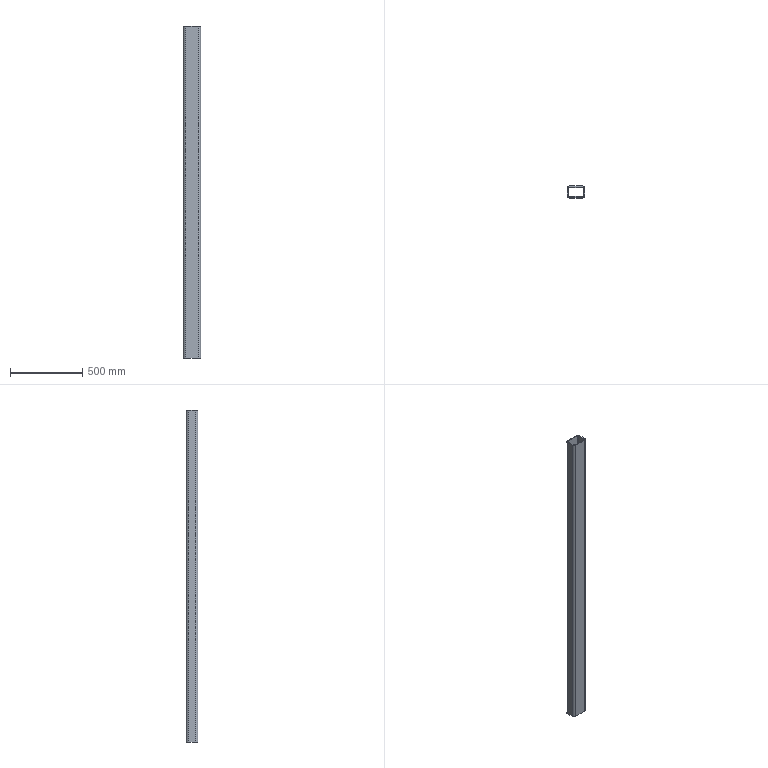Component | SolidWorks | ST60-04-1 | 1 solid | 18 faces | box 120 x 80 x 2300 mm | volume 6392127 mm3 | plane 10 | cylinder 8 | commonest cylinder face diameters 32 x4 16 x4
build123d program:
from build123d import *

# Parameters (mm, degrees)
RECTANGULAR_TUBE_120_X_80_X_8_1_DEPTH = 2300


with BuildPart() as part:
    # Sketch1 → Rectangular Tube 120 X 80 X 8_1 (new body)
    with BuildSketch(Plane.YZ):
        with BuildLine():
            Line((-24, -60), (24, -60))
            ThreePointArc((24, -60), (35.314, -55.314), (40, -44))
            Line((40, -44), (40, 44))
            ThreePointArc((40, 44), (35.314, 55.314), (24, 60))
            Line((24, 60), (-24, 60))
            ThreePointArc((-24, 60), (-35.314, 55.314), (-40, 44))
            Line((-40, 44), (-40, -44))
            ThreePointArc((-40, -44), (-35.314, -55.314), (-24, -60))
        make_face()
        with BuildLine():
            Line((-24, -52), (24, -52))
            ThreePointArc((24, -52), (29.657, -49.657), (32, -44))
            Line((32, -44), (32, 44))
            ThreePointArc((32, 44), (29.657, 49.657), (24, 52))
            Line((24, 52), (-24, 52))
            ThreePointArc((-24, 52), (-29.657, 49.657), (-32, 44))
            Line((-32, 44), (-32, -44))
            ThreePointArc((-32, -44), (-29.657, -49.657), (-24, -52))
        make_face(mode=Mode.SUBTRACT)
    extrude(amount=RECTANGULAR_TUBE_120_X_80_X_8_1_DEPTH)


solid = part.part

# Placed as in the assembly
solid = solid.moved(Location((592.993, -4.546, -60), (0, 90, 0)))
STEP:
#1=COLOUR_RGB('',0.7922,0.8196,0.9333);
#2=FILL_AREA_STYLE_COLOUR('',#1);
#3=FILL_AREA_STYLE('',(#2));
#4=SURFACE_STYLE_FILL_AREA(#3);
#5=SURFACE_SIDE_STYLE('',(#4));
#6=SURFACE_STYLE_USAGE(.BOTH.,#5);
#7=PRESENTATION_STYLE_ASSIGNMENT((#6));
#8=CARTESIAN_POINT('',(21.614,1.396,-92.913));
#9=VERTEX_POINT('',#8);
#10=CARTESIAN_POINT('',(20.984,0.7659,-92.913));
#11=VERTEX_POINT('',#10);
#12=CARTESIAN_POINT('',(21.614,0.7659,-92.913));
#13=DIRECTION('',(0.,0.,1.));
#14=DIRECTION('',(1.,0.,0.));
#15=AXIS2_PLACEMENT_3D('',#12,#13,#14);
#16=CIRCLE('',#15,0.6299);
#17=EDGE_CURVE('',#9,#11,#16,.T.);
#18=ORIENTED_EDGE('',*,*,#17,.T.);
#19=CARTESIAN_POINT('',(20.984,0.7659,-2.362));
#20=VERTEX_POINT('',#19);
#21=CARTESIAN_POINT('',(20.984,0.7659,-2.362));
#22=DIRECTION('',(0.,0.,-1.));
#23=VECTOR('',#22,39.37);
#24=LINE('',#21,#23);
#25=EDGE_CURVE('',#20,#11,#24,.T.);
#26=ORIENTED_EDGE('',*,*,#25,.F.);
#27=CARTESIAN_POINT('',(21.614,1.396,-2.362));
#28=VERTEX_POINT('',#27);
#29=CARTESIAN_POINT('',(21.614,0.7659,-2.362));
#30=DIRECTION('',(0.,0.,1.));
#31=DIRECTION('',(1.,0.,0.));
#32=AXIS2_PLACEMENT_3D('',#29,#30,#31);
#33=CIRCLE('',#32,0.6299);
#34=EDGE_CURVE('',#28,#20,#33,.T.);
#35=ORIENTED_EDGE('',*,*,#34,.F.);
#36=CARTESIAN_POINT('',(21.614,1.396,-2.362));
#37=DIRECTION('',(0.,0.,-1.));
#38=VECTOR('',#37,39.37);
#39=LINE('',#36,#38);
#40=EDGE_CURVE('',#28,#9,#39,.T.);
#41=ORIENTED_EDGE('',*,*,#40,.T.);
#42=EDGE_LOOP('',(#18,#26,#35,#41));
#43=FACE_OUTER_BOUND('',#42,.T.);
#44=CARTESIAN_POINT('',(21.614,0.7659,-2.362));
#45=DIRECTION('',(0.,0.,-1.));
#46=DIRECTION('',(-1.,0.,0.));
#47=AXIS2_PLACEMENT_3D('',#44,#45,#46);
#48=CYLINDRICAL_SURFACE('',#47,0.6299);
#49=ADVANCED_FACE('',(#43),#48,.T.);
#50=CARTESIAN_POINT('',(20.984,-1.124,-92.913));
#51=VERTEX_POINT('',#50);
#52=CARTESIAN_POINT('',(20.984,0.7659,-92.913));
#53=DIRECTION('',(0.,-1.,0.));
#54=VECTOR('',#53,39.37);
#55=LINE('',#52,#54);
#56=EDGE_CURVE('',#11,#51,#55,.T.);
#57=ORIENTED_EDGE('',*,*,#56,.T.);
#58=CARTESIAN_POINT('',(20.984,-1.124,-2.362));
#59=VERTEX_POINT('',#58);
#60=CARTESIAN_POINT('',(20.984,-1.124,-2.362));
#61=DIRECTION('',(0.,0.,-1.));
#62=VECTOR('',#61,39.37);
#63=LINE('',#60,#62);
#64=EDGE_CURVE('',#59,#51,#63,.T.);
#65=ORIENTED_EDGE('',*,*,#64,.F.);
#66=CARTESIAN_POINT('',(20.984,0.7659,-2.362));
#67=DIRECTION('',(0.,-1.,0.));
#68=VECTOR('',#67,39.37);
#69=LINE('',#66,#68);
#70=EDGE_CURVE('',#20,#59,#69,.T.);
#71=ORIENTED_EDGE('',*,*,#70,.F.);
#72=ORIENTED_EDGE('',*,*,#25,.T.);
#73=EDGE_LOOP('',(#57,#65,#71,#72));
#74=FACE_OUTER_BOUND('',#73,.T.);
#75=CARTESIAN_POINT('',(20.984,0.7659,-2.362));
#76=DIRECTION('',(1.,0.,0.));
#77=DIRECTION('',(0.,0.,-1.));
#78=AXIS2_PLACEMENT_3D('',#75,#76,#77);
#79=PLANE('',#78);
#80=ADVANCED_FACE('',(#74),#79,.F.);
#81=CARTESIAN_POINT('',(21.614,-1.754,-92.913));
#82=VERTEX_POINT('',#81);
#83=CARTESIAN_POINT('',(21.614,-1.124,-92.913));
#84=DIRECTION('',(0.,0.,1.));
#85=DIRECTION('',(1.,0.,0.));
#86=AXIS2_PLACEMENT_3D('',#83,#84,#85);
#87=CIRCLE('',#86,0.6299);
#88=EDGE_CURVE('',#51,#82,#87,.T.);
#89=ORIENTED_EDGE('',*,*,#88,.T.);
#90=CARTESIAN_POINT('',(21.614,-1.754,-2.362));
#91=VERTEX_POINT('',#90);
#92=CARTESIAN_POINT('',(21.614,-1.754,-2.362));
#93=DIRECTION('',(0.,0.,-1.));
#94=VECTOR('',#93,39.37);
#95=LINE('',#92,#94);
#96=EDGE_CURVE('',#91,#82,#95,.T.);
#97=ORIENTED_EDGE('',*,*,#96,.F.);
#98=CARTESIAN_POINT('',(21.614,-1.124,-2.362));
#99=DIRECTION('',(0.,0.,1.));
#100=DIRECTION('',(1.,0.,0.));
#101=AXIS2_PLACEMENT_3D('',#98,#99,#100);
#102=CIRCLE('',#101,0.6299);
#103=EDGE_CURVE('',#59,#91,#102,.T.);
#104=ORIENTED_EDGE('',*,*,#103,.F.);
#105=ORIENTED_EDGE('',*,*,#64,.T.);
#106=EDGE_LOOP('',(#89,#97,#104,#105));
#107=FACE_OUTER_BOUND('',#106,.T.);
#108=CARTESIAN_POINT('',(21.614,-1.124,-2.362));
#109=DIRECTION('',(0.,0.,-1.));
#110=DIRECTION('',(-1.,0.,0.));
#111=AXIS2_PLACEMENT_3D('',#108,#109,#110);
#112=CYLINDRICAL_SURFACE('',#111,0.6299);
#113=ADVANCED_FACE('',(#107),#112,.T.);
#114=CARTESIAN_POINT('',(25.078,-1.754,-92.913));
#115=VERTEX_POINT('',#114);
#116=CARTESIAN_POINT('',(25.078,-1.754,-92.913));
#117=DIRECTION('',(1.,0.,0.));
#118=VECTOR('',#117,39.37);
#119=LINE('',#116,#118);
#120=EDGE_CURVE('',#82,#115,#119,.T.);
#121=ORIENTED_EDGE('',*,*,#120,.T.);
#122=CARTESIAN_POINT('',(25.078,-1.754,-2.362));
#123=VERTEX_POINT('',#122);
#124=CARTESIAN_POINT('',(25.078,-1.754,-2.362));
#125=DIRECTION('',(0.,0.,-1.));
#126=VECTOR('',#125,39.37);
#127=LINE('',#124,#126);
#128=EDGE_CURVE('',#123,#115,#127,.T.);
#129=ORIENTED_EDGE('',*,*,#128,.F.);
#130=CARTESIAN_POINT('',(25.078,-1.754,-2.362));
#131=DIRECTION('',(1.,0.,0.));
#132=VECTOR('',#131,39.37);
#133=LINE('',#130,#132);
#134=EDGE_CURVE('',#91,#123,#133,.T.);
#135=ORIENTED_EDGE('',*,*,#134,.F.);
#136=ORIENTED_EDGE('',*,*,#96,.T.);
#137=EDGE_LOOP('',(#121,#129,#135,#136));
#138=FACE_OUTER_BOUND('',#137,.T.);
#139=CARTESIAN_POINT('',(25.078,-1.754,-2.362));
#140=DIRECTION('',(0.,1.,0.));
#141=DIRECTION('',(-1.,0.,0.));
#142=AXIS2_PLACEMENT_3D('',#139,#140,#141);
#143=PLANE('',#142);
#144=ADVANCED_FACE('',(#138),#143,.F.);
#145=CARTESIAN_POINT('',(25.708,-1.124,-92.913));
#146=VERTEX_POINT('',#145);
#147=CARTESIAN_POINT('',(25.078,-1.124,-92.913));
#148=DIRECTION('',(0.,0.,1.));
#149=DIRECTION('',(1.,0.,0.));
#150=AXIS2_PLACEMENT_3D('',#147,#148,#149);
#151=CIRCLE('',#150,0.6299);
#152=EDGE_CURVE('',#115,#146,#151,.T.);
#153=ORIENTED_EDGE('',*,*,#152,.T.);
#154=CARTESIAN_POINT('',(25.708,-1.124,-2.362));
#155=VERTEX_POINT('',#154);
#156=CARTESIAN_POINT('',(25.708,-1.124,-2.362));
#157=DIRECTION('',(0.,0.,-1.));
#158=VECTOR('',#157,39.37);
#159=LINE('',#156,#158);
#160=EDGE_CURVE('',#155,#146,#159,.T.);
#161=ORIENTED_EDGE('',*,*,#160,.F.);
#162=CARTESIAN_POINT('',(25.078,-1.124,-2.362));
#163=DIRECTION('',(0.,0.,1.));
#164=DIRECTION('',(1.,0.,0.));
#165=AXIS2_PLACEMENT_3D('',#162,#163,#164);
#166=CIRCLE('',#165,0.6299);
#167=EDGE_CURVE('',#123,#155,#166,.T.);
#168=ORIENTED_EDGE('',*,*,#167,.F.);
#169=ORIENTED_EDGE('',*,*,#128,.T.);
#170=EDGE_LOOP('',(#153,#161,#168,#169));
#171=FACE_OUTER_BOUND('',#170,.T.);
#172=CARTESIAN_POINT('',(25.078,-1.124,-2.362));
#173=DIRECTION('',(0.,0.,-1.));
#174=DIRECTION('',(-1.,0.,0.));
#175=AXIS2_PLACEMENT_3D('',#172,#173,#174);
#176=CYLINDRICAL_SURFACE('',#175,0.6299);
#177=ADVANCED_FACE('',(#171),#176,.T.);
#178=CARTESIAN_POINT('',(25.708,0.7659,-92.913));
#179=VERTEX_POINT('',#178);
#180=CARTESIAN_POINT('',(25.708,-1.124,-92.913));
#181=DIRECTION('',(0.,1.,0.));
#182=VECTOR('',#181,39.37);
#183=LINE('',#180,#182);
#184=EDGE_CURVE('',#146,#179,#183,.T.);
#185=ORIENTED_EDGE('',*,*,#184,.T.);
#186=CARTESIAN_POINT('',(25.708,0.7659,-2.362));
#187=VERTEX_POINT('',#186);
#188=CARTESIAN_POINT('',(25.708,0.7659,-2.362));
#189=DIRECTION('',(0.,0.,-1.));
#190=VECTOR('',#189,39.37);
#191=LINE('',#188,#190);
#192=EDGE_CURVE('',#187,#179,#191,.T.);
#193=ORIENTED_EDGE('',*,*,#192,.F.);
#194=CARTESIAN_POINT('',(25.708,-1.124,-2.362));
#195=DIRECTION('',(0.,1.,0.));
#196=VECTOR('',#195,39.37);
#197=LINE('',#194,#196);
#198=EDGE_CURVE('',#155,#187,#197,.T.);
#199=ORIENTED_EDGE('',*,*,#198,.F.);
#200=ORIENTED_EDGE('',*,*,#160,.T.);
#201=EDGE_LOOP('',(#185,#193,#199,#200));
#202=FACE_OUTER_BOUND('',#201,.T.);
#203=CARTESIAN_POINT('',(25.708,-1.124,-2.362));
#204=DIRECTION('',(-1.,0.,0.));
#205=DIRECTION('',(0.,0.,1.));
#206=AXIS2_PLACEMENT_3D('',#203,#204,#205);
#207=PLANE('',#206);
#208=ADVANCED_FACE('',(#202),#207,.F.);
#209=CARTESIAN_POINT('',(25.078,1.396,-92.913));
#210=VERTEX_POINT('',#209);
#211=CARTESIAN_POINT('',(25.078,0.7659,-92.913));
#212=DIRECTION('',(0.,0.,1.));
#213=DIRECTION('',(1.,0.,0.));
#214=AXIS2_PLACEMENT_3D('',#211,#212,#213);
#215=CIRCLE('',#214,0.6299);
#216=EDGE_CURVE('',#179,#210,#215,.T.);
#217=ORIENTED_EDGE('',*,*,#216,.T.);
#218=CARTESIAN_POINT('',(25.078,1.396,-2.362));
#219=VERTEX_POINT('',#218);
#220=CARTESIAN_POINT('',(25.078,1.396,-2.362));
#221=DIRECTION('',(0.,0.,-1.));
#222=VECTOR('',#221,39.37);
#223=LINE('',#220,#222);
#224=EDGE_CURVE('',#219,#210,#223,.T.);
#225=ORIENTED_EDGE('',*,*,#224,.F.);
#226=CARTESIAN_POINT('',(25.078,0.7659,-2.362));
#227=DIRECTION('',(0.,0.,1.));
#228=DIRECTION('',(1.,0.,0.));
#229=AXIS2_PLACEMENT_3D('',#226,#227,#228);
#230=CIRCLE('',#229,0.6299);
#231=EDGE_CURVE('',#187,#219,#230,.T.);
#232=ORIENTED_EDGE('',*,*,#231,.F.);
#233=ORIENTED_EDGE('',*,*,#192,.T.);
#234=EDGE_LOOP('',(#217,#225,#232,#233));
#235=FACE_OUTER_BOUND('',#234,.T.);
#236=CARTESIAN_POINT('',(25.078,0.7659,-2.362));
#237=DIRECTION('',(0.,0.,-1.));
#238=DIRECTION('',(-1.,0.,0.));
#239=AXIS2_PLACEMENT_3D('',#236,#237,#238);
#240=CYLINDRICAL_SURFACE('',#239,0.6299);
#241=ADVANCED_FACE('',(#235),#240,.T.);
#242=CARTESIAN_POINT('',(21.299,-1.124,-92.913));
#243=VERTEX_POINT('',#242);
#244=CARTESIAN_POINT('',(21.614,-1.439,-92.913));
#245=VERTEX_POINT('',#244);
#246=CARTESIAN_POINT('',(21.614,-1.124,-92.913));
#247=DIRECTION('',(0.,0.,1.));
#248=DIRECTION('',(1.,0.,0.));
#249=AXIS2_PLACEMENT_3D('',#246,#247,#248);
#250=CIRCLE('',#249,0.315);
#251=EDGE_CURVE('',#243,#245,#250,.T.);
#252=ORIENTED_EDGE('',*,*,#251,.F.);
#253=CARTESIAN_POINT('',(21.299,-1.124,-2.362));
#254=VERTEX_POINT('',#253);
#255=CARTESIAN_POINT('',(21.299,-1.124,-2.362));
#256=DIRECTION('',(0.,0.,-1.));
#257=VECTOR('',#256,39.37);
#258=LINE('',#255,#257);
#259=EDGE_CURVE('',#254,#243,#258,.T.);
#260=ORIENTED_EDGE('',*,*,#259,.F.);
#261=CARTESIAN_POINT('',(21.614,-1.439,-2.362));
#262=VERTEX_POINT('',#261);
#263=CARTESIAN_POINT('',(21.614,-1.124,-2.362));
#264=DIRECTION('',(0.,0.,1.));
#265=DIRECTION('',(1.,0.,0.));
#266=AXIS2_PLACEMENT_3D('',#263,#264,#265);
#267=CIRCLE('',#266,0.315);
#268=EDGE_CURVE('',#254,#262,#267,.T.);
#269=ORIENTED_EDGE('',*,*,#268,.T.);
#270=CARTESIAN_POINT('',(21.614,-1.439,-2.362));
#271=DIRECTION('',(0.,0.,-1.));
#272=VECTOR('',#271,39.37);
#273=LINE('',#270,#272);
#274=EDGE_CURVE('',#262,#245,#273,.T.);
#275=ORIENTED_EDGE('',*,*,#274,.T.);
#276=EDGE_LOOP('',(#252,#260,#269,#275));
#277=FACE_OUTER_BOUND('',#276,.T.);
#278=CARTESIAN_POINT('',(21.614,-1.124,-2.362));
#279=DIRECTION('',(0.,0.,-1.));
#280=DIRECTION('',(-1.,0.,0.));
#281=AXIS2_PLACEMENT_3D('',#278,#279,#280);
#282=CYLINDRICAL_SURFACE('',#281,0.315);
#283=ADVANCED_FACE('',(#277),#282,.F.);
#284=CARTESIAN_POINT('',(21.299,0.7659,-92.913));
#285=VERTEX_POINT('',#284);
#286=CARTESIAN_POINT('',(21.299,0.7659,-92.913));
#287=DIRECTION('',(0.,-1.,0.));
#288=VECTOR('',#287,39.37);
#289=LINE('',#286,#288);
#290=EDGE_CURVE('',#285,#243,#289,.T.);
#291=ORIENTED_EDGE('',*,*,#290,.F.);
#292=CARTESIAN_POINT('',(21.299,0.7659,-2.362));
#293=VERTEX_POINT('',#292);
#294=CARTESIAN_POINT('',(21.299,0.7659,-2.362));
#295=DIRECTION('',(0.,0.,-1.));
#296=VECTOR('',#295,39.37);
#297=LINE('',#294,#296);
#298=EDGE_CURVE('',#293,#285,#297,.T.);
#299=ORIENTED_EDGE('',*,*,#298,.F.);
#300=CARTESIAN_POINT('',(21.299,0.7659,-2.362));
#301=DIRECTION('',(0.,-1.,0.));
#302=VECTOR('',#301,39.37);
#303=LINE('',#300,#302);
#304=EDGE_CURVE('',#293,#254,#303,.T.);
#305=ORIENTED_EDGE('',*,*,#304,.T.);
#306=ORIENTED_EDGE('',*,*,#259,.T.);
#307=EDGE_LOOP('',(#291,#299,#305,#306));
#308=FACE_OUTER_BOUND('',#307,.T.);
#309=CARTESIAN_POINT('',(21.299,0.7659,-2.362));
#310=DIRECTION('',(1.,0.,0.));
#311=DIRECTION('',(0.,0.,-1.));
#312=AXIS2_PLACEMENT_3D('',#309,#310,#311);
#313=PLANE('',#312);
#314=ADVANCED_FACE('',(#308),#313,.T.);
#315=CARTESIAN_POINT('',(21.614,1.081,-92.913));
#316=VERTEX_POINT('',#315);
#317=CARTESIAN_POINT('',(21.614,0.7659,-92.913));
#318=DIRECTION('',(0.,0.,1.));
#319=DIRECTION('',(1.,0.,0.));
#320=AXIS2_PLACEMENT_3D('',#317,#318,#319);
#321=CIRCLE('',#320,0.315);
#322=EDGE_CURVE('',#316,#285,#321,.T.);
#323=ORIENTED_EDGE('',*,*,#322,.F.);
#324=CARTESIAN_POINT('',(21.614,1.081,-2.362));
#325=VERTEX_POINT('',#324);
#326=CARTESIAN_POINT('',(21.614,1.081,-2.362));
#327=DIRECTION('',(0.,0.,-1.));
#328=VECTOR('',#327,39.37);
#329=LINE('',#326,#328);
#330=EDGE_CURVE('',#325,#316,#329,.T.);
#331=ORIENTED_EDGE('',*,*,#330,.F.);
#332=CARTESIAN_POINT('',(21.614,0.7659,-2.362));
#333=DIRECTION('',(0.,0.,1.));
#334=DIRECTION('',(1.,0.,0.));
#335=AXIS2_PLACEMENT_3D('',#332,#333,#334);
#336=CIRCLE('',#335,0.315);
#337=EDGE_CURVE('',#325,#293,#336,.T.);
#338=ORIENTED_EDGE('',*,*,#337,.T.);
#339=ORIENTED_EDGE('',*,*,#298,.T.);
#340=EDGE_LOOP('',(#323,#331,#338,#339));
#341=FACE_OUTER_BOUND('',#340,.T.);
#342=CARTESIAN_POINT('',(21.614,0.7659,-2.362));
#343=DIRECTION('',(0.,0.,-1.));
#344=DIRECTION('',(-1.,0.,0.));
#345=AXIS2_PLACEMENT_3D('',#342,#343,#344);
#346=CYLINDRICAL_SURFACE('',#345,0.315);
#347=ADVANCED_FACE('',(#341),#346,.F.);
#348=CARTESIAN_POINT('',(25.078,1.081,-92.913));
#349=VERTEX_POINT('',#348);
#350=CARTESIAN_POINT('',(21.614,1.081,-92.913));
#351=DIRECTION('',(-1.,0.,0.));
#352=VECTOR('',#351,39.37);
#353=LINE('',#350,#352);
#354=EDGE_CURVE('',#349,#316,#353,.T.);
#355=ORIENTED_EDGE('',*,*,#354,.F.);
#356=CARTESIAN_POINT('',(25.078,1.081,-2.362));
#357=VERTEX_POINT('',#356);
#358=CARTESIAN_POINT('',(25.078,1.081,-2.362));
#359=DIRECTION('',(0.,0.,-1.));
#360=VECTOR('',#359,39.37);
#361=LINE('',#358,#360);
#362=EDGE_CURVE('',#357,#349,#361,.T.);
#363=ORIENTED_EDGE('',*,*,#362,.F.);
#364=CARTESIAN_POINT('',(21.614,1.081,-2.362));
#365=DIRECTION('',(-1.,0.,0.));
#366=VECTOR('',#365,39.37);
#367=LINE('',#364,#366);
#368=EDGE_CURVE('',#357,#325,#367,.T.);
#369=ORIENTED_EDGE('',*,*,#368,.T.);
#370=ORIENTED_EDGE('',*,*,#330,.T.);
#371=EDGE_LOOP('',(#355,#363,#369,#370));
#372=FACE_OUTER_BOUND('',#371,.T.);
#373=CARTESIAN_POINT('',(21.614,1.081,-2.362));
#374=DIRECTION('',(0.,-1.,0.));
#375=DIRECTION('',(1.,0.,0.));
#376=AXIS2_PLACEMENT_3D('',#373,#374,#375);
#377=PLANE('',#376);
#378=ADVANCED_FACE('',(#372),#377,.T.);
#379=CARTESIAN_POINT('',(25.393,0.7659,-92.913));
#380=VERTEX_POINT('',#379);
#381=CARTESIAN_POINT('',(25.078,0.7659,-92.913));
#382=DIRECTION('',(0.,0.,1.));
#383=DIRECTION('',(1.,0.,0.));
#384=AXIS2_PLACEMENT_3D('',#381,#382,#383);
#385=CIRCLE('',#384,0.315);
#386=EDGE_CURVE('',#380,#349,#385,.T.);
#387=ORIENTED_EDGE('',*,*,#386,.F.);
#388=CARTESIAN_POINT('',(25.393,0.7659,-2.362));
#389=VERTEX_POINT('',#388);
#390=CARTESIAN_POINT('',(25.393,0.7659,-2.362));
#391=DIRECTION('',(0.,0.,-1.));
#392=VECTOR('',#391,39.37);
#393=LINE('',#390,#392);
#394=EDGE_CURVE('',#389,#380,#393,.T.);
#395=ORIENTED_EDGE('',*,*,#394,.F.);
#396=CARTESIAN_POINT('',(25.078,0.7659,-2.362));
#397=DIRECTION('',(0.,0.,1.));
#398=DIRECTION('',(1.,0.,0.));
#399=AXIS2_PLACEMENT_3D('',#396,#397,#398);
#400=CIRCLE('',#399,0.315);
#401=EDGE_CURVE('',#389,#357,#400,.T.);
#402=ORIENTED_EDGE('',*,*,#401,.T.);
#403=ORIENTED_EDGE('',*,*,#362,.T.);
#404=EDGE_LOOP('',(#387,#395,#402,#403));
#405=FACE_OUTER_BOUND('',#404,.T.);
#406=CARTESIAN_POINT('',(25.078,0.7659,-2.362));
#407=DIRECTION('',(0.,0.,-1.));
#408=DIRECTION('',(-1.,0.,0.));
#409=AXIS2_PLACEMENT_3D('',#406,#407,#408);
#410=CYLINDRICAL_SURFACE('',#409,0.315);
#411=ADVANCED_FACE('',(#405),#410,.F.);
#412=CARTESIAN_POINT('',(25.393,-1.124,-92.913));
#413=VERTEX_POINT('',#412);
#414=CARTESIAN_POINT('',(25.393,-1.124,-92.913));
#415=DIRECTION('',(0.,1.,0.));
#416=VECTOR('',#415,39.37);
#417=LINE('',#414,#416);
#418=EDGE_CURVE('',#413,#380,#417,.T.);
#419=ORIENTED_EDGE('',*,*,#418,.F.);
#420=CARTESIAN_POINT('',(25.393,-1.124,-2.362));
#421=VERTEX_POINT('',#420);
#422=CARTESIAN_POINT('',(25.393,-1.124,-2.362));
#423=DIRECTION('',(0.,0.,-1.));
#424=VECTOR('',#423,39.37);
#425=LINE('',#422,#424);
#426=EDGE_CURVE('',#421,#413,#425,.T.);
#427=ORIENTED_EDGE('',*,*,#426,.F.);
#428=CARTESIAN_POINT('',(25.393,-1.124,-2.362));
#429=DIRECTION('',(0.,1.,0.));
#430=VECTOR('',#429,39.37);
#431=LINE('',#428,#430);
#432=EDGE_CURVE('',#421,#389,#431,.T.);
#433=ORIENTED_EDGE('',*,*,#432,.T.);
#434=ORIENTED_EDGE('',*,*,#394,.T.);
#435=EDGE_LOOP('',(#419,#427,#433,#434));
#436=FACE_OUTER_BOUND('',#435,.T.);
#437=CARTESIAN_POINT('',(25.393,-1.124,-2.362));
#438=DIRECTION('',(-1.,0.,0.));
#439=DIRECTION('',(0.,0.,1.));
#440=AXIS2_PLACEMENT_3D('',#437,#438,#439);
#441=PLANE('',#440);
#442=ADVANCED_FACE('',(#436),#441,.T.);
#443=CARTESIAN_POINT('',(25.078,-1.439,-92.913));
#444=VERTEX_POINT('',#443);
#445=CARTESIAN_POINT('',(25.078,-1.124,-92.913));
#446=DIRECTION('',(0.,0.,1.));
#447=DIRECTION('',(1.,0.,0.));
#448=AXIS2_PLACEMENT_3D('',#445,#446,#447);
#449=CIRCLE('',#448,0.315);
#450=EDGE_CURVE('',#444,#413,#449,.T.);
#451=ORIENTED_EDGE('',*,*,#450,.F.);
#452=CARTESIAN_POINT('',(25.078,-1.439,-2.362));
#453=VERTEX_POINT('',#452);
#454=CARTESIAN_POINT('',(25.078,-1.439,-2.362));
#455=DIRECTION('',(0.,0.,-1.));
#456=VECTOR('',#455,39.37);
#457=LINE('',#454,#456);
#458=EDGE_CURVE('',#453,#444,#457,.T.);
#459=ORIENTED_EDGE('',*,*,#458,.F.);
#460=CARTESIAN_POINT('',(25.078,-1.124,-2.362));
#461=DIRECTION('',(0.,0.,1.));
#462=DIRECTION('',(1.,0.,0.));
#463=AXIS2_PLACEMENT_3D('',#460,#461,#462);
#464=CIRCLE('',#463,0.315);
#465=EDGE_CURVE('',#453,#421,#464,.T.);
#466=ORIENTED_EDGE('',*,*,#465,.T.);
#467=ORIENTED_EDGE('',*,*,#426,.T.);
#468=EDGE_LOOP('',(#451,#459,#466,#467));
#469=FACE_OUTER_BOUND('',#468,.T.);
#470=CARTESIAN_POINT('',(25.078,-1.124,-2.362));
#471=DIRECTION('',(0.,0.,-1.));
#472=DIRECTION('',(-1.,0.,0.));
#473=AXIS2_PLACEMENT_3D('',#470,#471,#472);
#474=CYLINDRICAL_SURFACE('',#473,0.315);
#475=ADVANCED_FACE('',(#469),#474,.F.);
#476=CARTESIAN_POINT('',(25.078,-1.439,-92.913));
#477=DIRECTION('',(1.,0.,0.));
#478=VECTOR('',#477,39.37);
#479=LINE('',#476,#478);
#480=EDGE_CURVE('',#245,#444,#479,.T.);
#481=ORIENTED_EDGE('',*,*,#480,.F.);
#482=ORIENTED_EDGE('',*,*,#274,.F.);
#483=CARTESIAN_POINT('',(25.078,-1.439,-2.362));
#484=DIRECTION('',(1.,0.,0.));
#485=VECTOR('',#484,39.37);
#486=LINE('',#483,#485);
#487=EDGE_CURVE('',#262,#453,#486,.T.);
#488=ORIENTED_EDGE('',*,*,#487,.T.);
#489=ORIENTED_EDGE('',*,*,#458,.T.);
#490=EDGE_LOOP('',(#481,#482,#488,#489));
#491=FACE_OUTER_BOUND('',#490,.T.);
#492=CARTESIAN_POINT('',(25.078,-1.439,-2.362));
#493=DIRECTION('',(0.,1.,0.));
#494=DIRECTION('',(-1.,0.,0.));
#495=AXIS2_PLACEMENT_3D('',#492,#493,#494);
#496=PLANE('',#495);
#497=ADVANCED_FACE('',(#491),#496,.T.);
#498=CARTESIAN_POINT('',(21.614,1.396,-92.913));
#499=DIRECTION('',(-1.,0.,0.));
#500=VECTOR('',#499,39.37);
#501=LINE('',#498,#500);
#502=EDGE_CURVE('',#210,#9,#501,.T.);
#503=ORIENTED_EDGE('',*,*,#502,.T.);
#504=ORIENTED_EDGE('',*,*,#40,.F.);
#505=CARTESIAN_POINT('',(21.614,1.396,-2.362));
#506=DIRECTION('',(-1.,0.,0.));
#507=VECTOR('',#506,39.37);
#508=LINE('',#505,#507);
#509=EDGE_CURVE('',#219,#28,#508,.T.);
#510=ORIENTED_EDGE('',*,*,#509,.F.);
#511=ORIENTED_EDGE('',*,*,#224,.T.);
#512=EDGE_LOOP('',(#503,#504,#510,#511));
#513=FACE_OUTER_BOUND('',#512,.T.);
#514=CARTESIAN_POINT('',(21.614,1.396,-2.362));
#515=DIRECTION('',(0.,-1.,0.));
#516=DIRECTION('',(1.,0.,0.));
#517=AXIS2_PLACEMENT_3D('',#514,#515,#516);
#518=PLANE('',#517);
#519=ADVANCED_FACE('',(#513),#518,.F.);
#520=ORIENTED_EDGE('',*,*,#268,.F.);
#521=ORIENTED_EDGE('',*,*,#304,.F.);
#522=ORIENTED_EDGE('',*,*,#337,.F.);
#523=ORIENTED_EDGE('',*,*,#368,.F.);
#524=ORIENTED_EDGE('',*,*,#401,.F.);
#525=ORIENTED_EDGE('',*,*,#432,.F.);
#526=ORIENTED_EDGE('',*,*,#465,.F.);
#527=ORIENTED_EDGE('',*,*,#487,.F.);
#528=EDGE_LOOP('',(#520,#521,#522,#523,#524,#525,#526,#527));
#529=FACE_BOUND('',#528,.T.);
#530=ORIENTED_EDGE('',*,*,#34,.T.);
#531=ORIENTED_EDGE('',*,*,#70,.T.);
#532=ORIENTED_EDGE('',*,*,#103,.T.);
#533=ORIENTED_EDGE('',*,*,#134,.T.);
#534=ORIENTED_EDGE('',*,*,#167,.T.);
#535=ORIENTED_EDGE('',*,*,#198,.T.);
#536=ORIENTED_EDGE('',*,*,#231,.T.);
#537=ORIENTED_EDGE('',*,*,#509,.T.);
#538=EDGE_LOOP('',(#530,#531,#532,#533,#534,#535,#536,#537));
#539=FACE_OUTER_BOUND('',#538,.T.);
#540=CARTESIAN_POINT('',(21.614,0.7659,-2.362));
#541=DIRECTION('',(0.,0.,1.));
#542=DIRECTION('',(1.,0.,0.));
#543=AXIS2_PLACEMENT_3D('',#540,#541,#542);
#544=PLANE('',#543);
#545=ADVANCED_FACE('',(#529,#539),#544,.T.);
#546=ORIENTED_EDGE('',*,*,#251,.T.);
#547=ORIENTED_EDGE('',*,*,#480,.T.);
#548=ORIENTED_EDGE('',*,*,#450,.T.);
#549=ORIENTED_EDGE('',*,*,#418,.T.);
#550=ORIENTED_EDGE('',*,*,#386,.T.);
#551=ORIENTED_EDGE('',*,*,#354,.T.);
#552=ORIENTED_EDGE('',*,*,#322,.T.);
#553=ORIENTED_EDGE('',*,*,#290,.T.);
#554=EDGE_LOOP('',(#546,#547,#548,#549,#550,#551,#552,#553));
#555=FACE_BOUND('',#554,.T.);
#556=ORIENTED_EDGE('',*,*,#17,.F.);
#557=ORIENTED_EDGE('',*,*,#502,.F.);
#558=ORIENTED_EDGE('',*,*,#216,.F.);
#559=ORIENTED_EDGE('',*,*,#184,.F.);
#560=ORIENTED_EDGE('',*,*,#152,.F.);
#561=ORIENTED_EDGE('',*,*,#120,.F.);
#562=ORIENTED_EDGE('',*,*,#88,.F.);
#563=ORIENTED_EDGE('',*,*,#56,.F.);
#564=EDGE_LOOP('',(#556,#557,#558,#559,#560,#561,#562,#563));
#565=FACE_OUTER_BOUND('',#564,.T.);
#566=CARTESIAN_POINT('',(21.614,0.7659,-92.913));
#567=DIRECTION('',(0.,0.,1.));
#568=DIRECTION('',(1.,0.,0.));
#569=AXIS2_PLACEMENT_3D('',#566,#567,#568);
#570=PLANE('',#569);
#571=ADVANCED_FACE('',(#555,#565),#570,.F.);
#572=CLOSED_SHELL('',(#49,#80,#113,#144,#177,#208,#241,#283,#314,#347,#378,#411,#442,#475,#497,#519,#545,#571));
#573=MANIFOLD_SOLID_BREP('',#572);
#574=STYLED_ITEM('',(#7),#573);
#575=(LENGTH_UNIT()NAMED_UNIT(*)SI_UNIT($,.METRE.));
#576=LENGTH_MEASURE_WITH_UNIT(LENGTH_MEASURE(0.0254),#575);
#577=DIMENSIONAL_EXPONENTS(1.,0.,0.,0.,0.,0.,0.);
#578=(CONVERSION_BASED_UNIT('',#576)LENGTH_UNIT()NAMED_UNIT(#577));
#579=UNCERTAINTY_MEASURE_WITH_UNIT(LENGTH_MEASURE(0.00001),#578,'','');
#580=(NAMED_UNIT(*)PLANE_ANGLE_UNIT()SI_UNIT($,.RADIAN.));
#581=(NAMED_UNIT(*)SI_UNIT($,.STERADIAN.)SOLID_ANGLE_UNIT());
#582=(GEOMETRIC_REPRESENTATION_CONTEXT(3)GLOBAL_UNCERTAINTY_ASSIGNED_CONTEXT((#579))GLOBAL_UNIT_ASSIGNED_CONTEXT((#578,#580,#581))REPRESENTATION_CONTEXT('',''));
#583=MECHANICAL_DESIGN_GEOMETRIC_PRESENTATION_REPRESENTATION('',(#574),#582);
#584=CARTESIAN_POINT('',(0.,0.,0.));
#585=DIRECTION('',(0.,0.,1.));
#586=DIRECTION('',(1.,0.,0.));
#587=AXIS2_PLACEMENT_3D('',#584,#585,#586);
#588=(LENGTH_UNIT()NAMED_UNIT(*)SI_UNIT($,.METRE.));
#589=LENGTH_MEASURE_WITH_UNIT(LENGTH_MEASURE(0.0254),#588);
#590=DIMENSIONAL_EXPONENTS(1.,0.,0.,0.,0.,0.,0.);
#591=(CONVERSION_BASED_UNIT('',#589)LENGTH_UNIT()NAMED_UNIT(#590));
#592=UNCERTAINTY_MEASURE_WITH_UNIT(LENGTH_MEASURE(0.00001),#591,'','');
#593=(NAMED_UNIT(*)PLANE_ANGLE_UNIT()SI_UNIT($,.RADIAN.));
#594=(NAMED_UNIT(*)SI_UNIT($,.STERADIAN.)SOLID_ANGLE_UNIT());
#595=(GEOMETRIC_REPRESENTATION_CONTEXT(3)GLOBAL_UNCERTAINTY_ASSIGNED_CONTEXT((#592))GLOBAL_UNIT_ASSIGNED_CONTEXT((#591,#593,#594))REPRESENTATION_CONTEXT('',''));
#596=ADVANCED_BREP_SHAPE_REPRESENTATION('',(#573,#587),#595);
#597=PRESENTATION_LAYER_ASSIGNMENT('','',(#574));